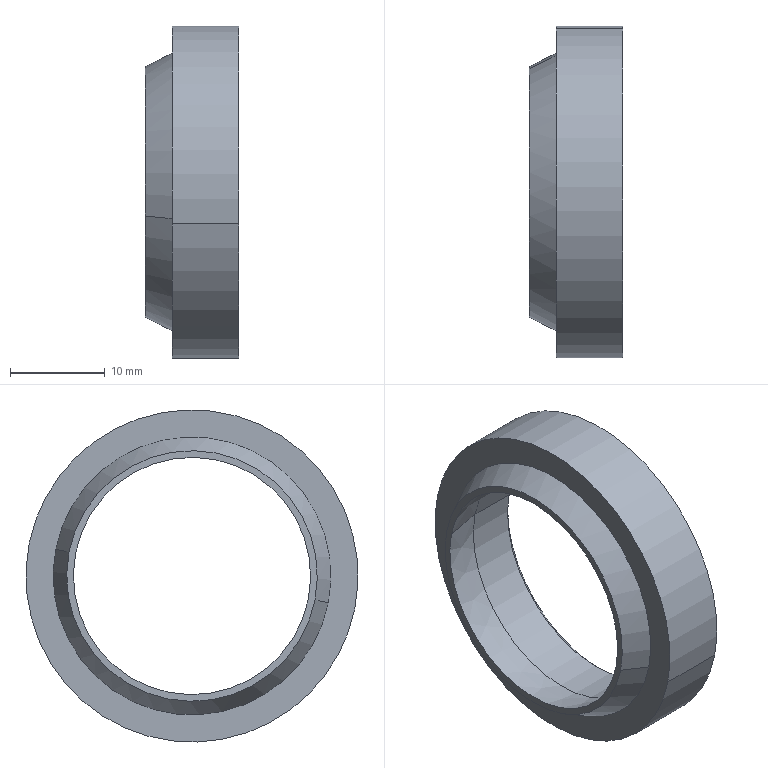Component | SolidWorks | GB_T10708.3-1989TypeBRubberDustSealFB20_35_7-1 | 1 solid | 13 faces | box 9.8 x 35 x 35 mm | volume 3185 mm3 | cone 6 | cylinder 4 | plane 3 | commonest cylinder face diameters 26.4 x2 35 x2
build123d program:
from build123d import *

# Parameters (mm, degrees)
CHAMFER1_SIZE = 0.5


with BuildPart() as part:
    # Sketch1 → Base-Revolve (revolve)
    with BuildSketch(Plane.XY, mode=Mode.PRIVATE) as base_revolve_sk:
        Polygon((12.5, 9.8), (13.2, 9.8), (14.633, 7), (17.5, 7), (17.5, 0), (13.2, 0), (13.2, 5.6), align=None)
    revolve(base_revolve_sk.sketch.rotate(Axis((0, 0, 0), (0, 1, 0)), 90), axis=Axis((0, 0, 0), (0, 1, 0)))

    # Chamfer1
    chamfer1_edges = [part.edges().sort_by_distance(p)[0] for p in [
        (0, 0, 13.2),
    ]]
    chamfer(chamfer1_edges, length=CHAMFER1_SIZE)


solid = part.part

# Placed as in the assembly
solid = solid.moved(Location((-465.364, 0, 0), (0, 0, 90)))
STEP:
#1=COLOUR_RGB('',0.7922,0.8196,0.9333);
#2=FILL_AREA_STYLE_COLOUR('',#1);
#3=FILL_AREA_STYLE('',(#2));
#4=SURFACE_STYLE_FILL_AREA(#3);
#5=SURFACE_SIDE_STYLE('',(#4));
#6=SURFACE_STYLE_USAGE(.BOTH.,#5);
#7=PRESENTATION_STYLE_ASSIGNMENT((#6));
#8=CARTESIAN_POINT('',(-18.341,-0.51,-0.09992));
#9=VERTEX_POINT('',#8);
#10=CARTESIAN_POINT('',(-18.341,0.51,0.09992));
#11=VERTEX_POINT('',#10);
#12=CARTESIAN_POINT('',(-18.341,0.,-0.));
#13=DIRECTION('',(1.,-0.,0.));
#14=DIRECTION('',(0.,0.9813,0.1923));
#15=AXIS2_PLACEMENT_3D('',#12,#13,#14);
#16=CIRCLE('',#15,0.5197);
#17=EDGE_CURVE('',#9,#11,#16,.T.);
#18=ORIENTED_EDGE('',*,*,#17,.F.);
#19=CARTESIAN_POINT('',(-18.321,-0.5293,-0.1037));
#20=VERTEX_POINT('',#19);
#21=CARTESIAN_POINT('',(-18.341,-0.51,-0.09992));
#22=DIRECTION('',(0.7071,-0.6939,-0.136));
#23=VECTOR('',#22,39.37);
#24=LINE('',#21,#23);
#25=EDGE_CURVE('',#9,#20,#24,.T.);
#26=ORIENTED_EDGE('',*,*,#25,.T.);
#27=CARTESIAN_POINT('',(-18.321,0.5293,0.1037));
#28=VERTEX_POINT('',#27);
#29=CARTESIAN_POINT('',(-18.321,0.,-0.));
#30=DIRECTION('',(-1.,0.,-0.));
#31=DIRECTION('',(0.,0.9813,0.1923));
#32=AXIS2_PLACEMENT_3D('',#29,#30,#31);
#33=CIRCLE('',#32,0.5394);
#34=EDGE_CURVE('',#28,#20,#33,.T.);
#35=ORIENTED_EDGE('',*,*,#34,.F.);
#36=CARTESIAN_POINT('',(-18.341,0.51,0.09992));
#37=DIRECTION('',(0.7071,0.6939,0.136));
#38=VECTOR('',#37,39.37);
#39=LINE('',#36,#38);
#40=EDGE_CURVE('',#11,#28,#39,.T.);
#41=ORIENTED_EDGE('',*,*,#40,.F.);
#42=EDGE_LOOP('',(#18,#26,#35,#41));
#43=FACE_OUTER_BOUND('',#42,.T.);
#44=CARTESIAN_POINT('',(-18.341,0.,-0.));
#45=DIRECTION('',(1.,-0.,0.));
#46=DIRECTION('',(0.,0.9813,0.1923));
#47=AXIS2_PLACEMENT_3D('',#44,#45,#46);
#48=CONICAL_SURFACE('',#47,0.5197,0.7854);
#49=ADVANCED_FACE('',(#43),#48,.F.);
#50=CARTESIAN_POINT('',(-18.542,-0.51,-0.09992));
#51=VERTEX_POINT('',#50);
#52=CARTESIAN_POINT('',(-18.542,0.51,0.09992));
#53=VERTEX_POINT('',#52);
#54=CARTESIAN_POINT('',(-18.542,0.,-0.));
#55=DIRECTION('',(1.,-0.,0.));
#56=DIRECTION('',(0.,0.9813,0.1923));
#57=AXIS2_PLACEMENT_3D('',#54,#55,#56);
#58=CIRCLE('',#57,0.5197);
#59=EDGE_CURVE('',#51,#53,#58,.T.);
#60=ORIENTED_EDGE('',*,*,#59,.F.);
#61=CARTESIAN_POINT('',(-18.321,-0.51,-0.09992));
#62=DIRECTION('',(1.,-0.,0.));
#63=VECTOR('',#62,39.37);
#64=LINE('',#61,#63);
#65=EDGE_CURVE('',#51,#9,#64,.T.);
#66=ORIENTED_EDGE('',*,*,#65,.T.);
#67=ORIENTED_EDGE('',*,*,#17,.T.);
#68=CARTESIAN_POINT('',(-18.321,0.51,0.09992));
#69=DIRECTION('',(1.,-0.,0.));
#70=VECTOR('',#69,39.37);
#71=LINE('',#68,#70);
#72=EDGE_CURVE('',#53,#11,#71,.T.);
#73=ORIENTED_EDGE('',*,*,#72,.F.);
#74=EDGE_LOOP('',(#60,#66,#67,#73));
#75=FACE_OUTER_BOUND('',#74,.T.);
#76=CARTESIAN_POINT('',(-18.321,0.,-0.));
#77=DIRECTION('',(1.,-0.,0.));
#78=DIRECTION('',(0.,0.9813,0.1923));
#79=AXIS2_PLACEMENT_3D('',#76,#77,#78);
#80=CYLINDRICAL_SURFACE('',#79,0.5197);
#81=ADVANCED_FACE('',(#75),#80,.F.);
#82=CARTESIAN_POINT('',(-18.597,0.6761,0.1325));
#83=VERTEX_POINT('',#82);
#84=CARTESIAN_POINT('',(-18.597,-0.6761,-0.1325));
#85=VERTEX_POINT('',#84);
#86=CARTESIAN_POINT('',(-18.597,0.,-0.));
#87=DIRECTION('',(1.,-0.,0.));
#88=DIRECTION('',(0.,0.9813,0.1923));
#89=AXIS2_PLACEMENT_3D('',#86,#87,#88);
#90=CIRCLE('',#89,0.689);
#91=EDGE_CURVE('',#83,#85,#90,.T.);
#92=ORIENTED_EDGE('',*,*,#91,.T.);
#93=CARTESIAN_POINT('',(-18.321,-0.6761,-0.1325));
#94=VERTEX_POINT('',#93);
#95=CARTESIAN_POINT('',(-18.321,-0.6761,-0.1325));
#96=DIRECTION('',(1.,-0.,0.));
#97=VECTOR('',#96,39.37);
#98=LINE('',#95,#97);
#99=EDGE_CURVE('',#85,#94,#98,.T.);
#100=ORIENTED_EDGE('',*,*,#99,.T.);
#101=CARTESIAN_POINT('',(-18.321,0.6761,0.1325));
#102=VERTEX_POINT('',#101);
#103=CARTESIAN_POINT('',(-18.321,0.,-0.));
#104=DIRECTION('',(1.,-0.,0.));
#105=DIRECTION('',(0.,0.9813,0.1923));
#106=AXIS2_PLACEMENT_3D('',#103,#104,#105);
#107=CIRCLE('',#106,0.689);
#108=EDGE_CURVE('',#102,#94,#107,.T.);
#109=ORIENTED_EDGE('',*,*,#108,.F.);
#110=CARTESIAN_POINT('',(-18.321,0.6761,0.1325));
#111=DIRECTION('',(1.,-0.,0.));
#112=VECTOR('',#111,39.37);
#113=LINE('',#110,#112);
#114=EDGE_CURVE('',#83,#102,#113,.T.);
#115=ORIENTED_EDGE('',*,*,#114,.F.);
#116=EDGE_LOOP('',(#92,#100,#109,#115));
#117=FACE_OUTER_BOUND('',#116,.T.);
#118=CARTESIAN_POINT('',(-18.321,0.,-0.));
#119=DIRECTION('',(1.,-0.,0.));
#120=DIRECTION('',(0.,0.9813,0.1923));
#121=AXIS2_PLACEMENT_3D('',#118,#119,#120);
#122=CYLINDRICAL_SURFACE('',#121,0.689);
#123=ADVANCED_FACE('',(#117),#122,.T.);
#124=CARTESIAN_POINT('',(-18.707,0.51,0.09992));
#125=VERTEX_POINT('',#124);
#126=CARTESIAN_POINT('',(-18.707,-0.51,-0.09992));
#127=VERTEX_POINT('',#126);
#128=CARTESIAN_POINT('',(-18.707,0.,-0.));
#129=DIRECTION('',(1.,-0.,0.));
#130=DIRECTION('',(0.,0.9813,0.1923));
#131=AXIS2_PLACEMENT_3D('',#128,#129,#130);
#132=CIRCLE('',#131,0.5197);
#133=EDGE_CURVE('',#125,#127,#132,.T.);
#134=ORIENTED_EDGE('',*,*,#133,.T.);
#135=CARTESIAN_POINT('',(-18.597,-0.5654,-0.1108));
#136=VERTEX_POINT('',#135);
#137=CARTESIAN_POINT('',(-18.597,-0.5654,-0.1108));
#138=DIRECTION('',(0.8901,-0.4472,-0.08761));
#139=VECTOR('',#138,39.37);
#140=LINE('',#137,#139);
#141=EDGE_CURVE('',#127,#136,#140,.T.);
#142=ORIENTED_EDGE('',*,*,#141,.T.);
#143=CARTESIAN_POINT('',(-18.597,0.5654,0.1108));
#144=VERTEX_POINT('',#143);
#145=CARTESIAN_POINT('',(-18.597,0.,-0.));
#146=DIRECTION('',(1.,-0.,0.));
#147=DIRECTION('',(0.,0.9813,0.1923));
#148=AXIS2_PLACEMENT_3D('',#145,#146,#147);
#149=CIRCLE('',#148,0.5761);
#150=EDGE_CURVE('',#144,#136,#149,.T.);
#151=ORIENTED_EDGE('',*,*,#150,.F.);
#152=CARTESIAN_POINT('',(-18.597,0.5654,0.1108));
#153=DIRECTION('',(0.8901,0.4472,0.08761));
#154=VECTOR('',#153,39.37);
#155=LINE('',#152,#154);
#156=EDGE_CURVE('',#125,#144,#155,.T.);
#157=ORIENTED_EDGE('',*,*,#156,.F.);
#158=EDGE_LOOP('',(#134,#142,#151,#157));
#159=FACE_OUTER_BOUND('',#158,.T.);
#160=CARTESIAN_POINT('',(-18.597,0.,-0.));
#161=DIRECTION('',(1.,-0.,0.));
#162=DIRECTION('',(0.,0.9813,0.1923));
#163=AXIS2_PLACEMENT_3D('',#160,#161,#162);
#164=CONICAL_SURFACE('',#163,0.5761,0.4731);
#165=ADVANCED_FACE('',(#159),#164,.T.);
#166=CARTESIAN_POINT('',(-18.707,-0.4829,-0.09462));
#167=VERTEX_POINT('',#166);
#168=CARTESIAN_POINT('',(-18.707,0.4829,0.09462));
#169=VERTEX_POINT('',#168);
#170=CARTESIAN_POINT('',(-18.707,0.,-0.));
#171=DIRECTION('',(1.,-0.,0.));
#172=DIRECTION('',(0.,0.9813,0.1923));
#173=AXIS2_PLACEMENT_3D('',#170,#171,#172);
#174=CIRCLE('',#173,0.4921);
#175=EDGE_CURVE('',#167,#169,#174,.T.);
#176=ORIENTED_EDGE('',*,*,#175,.F.);
#177=CARTESIAN_POINT('',(-18.707,-0.4829,-0.09462));
#178=DIRECTION('',(0.9864,-0.1613,-0.03161));
#179=VECTOR('',#178,39.37);
#180=LINE('',#177,#179);
#181=EDGE_CURVE('',#167,#51,#180,.T.);
#182=ORIENTED_EDGE('',*,*,#181,.T.);
#183=ORIENTED_EDGE('',*,*,#59,.T.);
#184=CARTESIAN_POINT('',(-18.707,0.4829,0.09462));
#185=DIRECTION('',(0.9864,0.1613,0.03161));
#186=VECTOR('',#185,39.37);
#187=LINE('',#184,#186);
#188=EDGE_CURVE('',#169,#53,#187,.T.);
#189=ORIENTED_EDGE('',*,*,#188,.F.);
#190=EDGE_LOOP('',(#176,#182,#183,#189));
#191=FACE_OUTER_BOUND('',#190,.T.);
#192=CARTESIAN_POINT('',(-18.707,0.,-0.));
#193=DIRECTION('',(1.,-0.,0.));
#194=DIRECTION('',(0.,0.9813,0.1923));
#195=AXIS2_PLACEMENT_3D('',#192,#193,#194);
#196=CONICAL_SURFACE('',#195,0.4921,0.1651);
#197=ADVANCED_FACE('',(#191),#196,.F.);
#198=ORIENTED_EDGE('',*,*,#181,.F.);
#199=CARTESIAN_POINT('',(-18.707,0.,-0.));
#200=DIRECTION('',(1.,-0.,0.));
#201=DIRECTION('',(0.,0.9813,0.1923));
#202=AXIS2_PLACEMENT_3D('',#199,#200,#201);
#203=CIRCLE('',#202,0.4921);
#204=EDGE_CURVE('',#169,#167,#203,.T.);
#205=ORIENTED_EDGE('',*,*,#204,.F.);
#206=ORIENTED_EDGE('',*,*,#188,.T.);
#207=CARTESIAN_POINT('',(-18.542,0.,-0.));
#208=DIRECTION('',(1.,-0.,0.));
#209=DIRECTION('',(0.,0.9813,0.1923));
#210=AXIS2_PLACEMENT_3D('',#207,#208,#209);
#211=CIRCLE('',#210,0.5197);
#212=EDGE_CURVE('',#53,#51,#211,.T.);
#213=ORIENTED_EDGE('',*,*,#212,.T.);
#214=EDGE_LOOP('',(#198,#205,#206,#213));
#215=FACE_OUTER_BOUND('',#214,.T.);
#216=CARTESIAN_POINT('',(-18.707,0.,-0.));
#217=DIRECTION('',(1.,-0.,0.));
#218=DIRECTION('',(0.,0.9813,0.1923));
#219=AXIS2_PLACEMENT_3D('',#216,#217,#218);
#220=CONICAL_SURFACE('',#219,0.4921,0.1651);
#221=ADVANCED_FACE('',(#215),#220,.F.);
#222=ORIENTED_EDGE('',*,*,#204,.T.);
#223=ORIENTED_EDGE('',*,*,#175,.T.);
#224=EDGE_LOOP('',(#222,#223));
#225=FACE_BOUND('',#224,.T.);
#226=ORIENTED_EDGE('',*,*,#133,.F.);
#227=CARTESIAN_POINT('',(-18.707,0.,-0.));
#228=DIRECTION('',(1.,-0.,0.));
#229=DIRECTION('',(0.,0.9813,0.1923));
#230=AXIS2_PLACEMENT_3D('',#227,#228,#229);
#231=CIRCLE('',#230,0.5197);
#232=EDGE_CURVE('',#127,#125,#231,.T.);
#233=ORIENTED_EDGE('',*,*,#232,.F.);
#234=EDGE_LOOP('',(#226,#233));
#235=FACE_OUTER_BOUND('',#234,.T.);
#236=CARTESIAN_POINT('',(-18.707,-0.09462,0.4829));
#237=DIRECTION('',(-1.,0.,-0.));
#238=DIRECTION('',(-0.,-0.9813,-0.1923));
#239=AXIS2_PLACEMENT_3D('',#236,#237,#238);
#240=PLANE('',#239);
#241=ADVANCED_FACE('',(#225,#235),#240,.T.);
#242=ORIENTED_EDGE('',*,*,#141,.F.);
#243=ORIENTED_EDGE('',*,*,#232,.T.);
#244=ORIENTED_EDGE('',*,*,#156,.T.);
#245=CARTESIAN_POINT('',(-18.597,0.,-0.));
#246=DIRECTION('',(1.,-0.,0.));
#247=DIRECTION('',(0.,0.9813,0.1923));
#248=AXIS2_PLACEMENT_3D('',#245,#246,#247);
#249=CIRCLE('',#248,0.5761);
#250=EDGE_CURVE('',#136,#144,#249,.T.);
#251=ORIENTED_EDGE('',*,*,#250,.F.);
#252=EDGE_LOOP('',(#242,#243,#244,#251));
#253=FACE_OUTER_BOUND('',#252,.T.);
#254=CARTESIAN_POINT('',(-18.597,0.,-0.));
#255=DIRECTION('',(1.,-0.,0.));
#256=DIRECTION('',(0.,0.9813,0.1923));
#257=AXIS2_PLACEMENT_3D('',#254,#255,#256);
#258=CONICAL_SURFACE('',#257,0.5761,0.4731);
#259=ADVANCED_FACE('',(#253),#258,.T.);
#260=ORIENTED_EDGE('',*,*,#150,.T.);
#261=ORIENTED_EDGE('',*,*,#250,.T.);
#262=EDGE_LOOP('',(#260,#261));
#263=FACE_BOUND('',#262,.T.);
#264=ORIENTED_EDGE('',*,*,#91,.F.);
#265=CARTESIAN_POINT('',(-18.597,0.,-0.));
#266=DIRECTION('',(1.,-0.,0.));
#267=DIRECTION('',(0.,0.9813,0.1923));
#268=AXIS2_PLACEMENT_3D('',#265,#266,#267);
#269=CIRCLE('',#268,0.689);
#270=EDGE_CURVE('',#85,#83,#269,.T.);
#271=ORIENTED_EDGE('',*,*,#270,.F.);
#272=EDGE_LOOP('',(#264,#271));
#273=FACE_OUTER_BOUND('',#272,.T.);
#274=CARTESIAN_POINT('',(-18.597,-0.1108,0.5654));
#275=DIRECTION('',(-1.,0.,-0.));
#276=DIRECTION('',(-0.,-0.9813,-0.1923));
#277=AXIS2_PLACEMENT_3D('',#274,#275,#276);
#278=PLANE('',#277);
#279=ADVANCED_FACE('',(#263,#273),#278,.T.);
#280=ORIENTED_EDGE('',*,*,#99,.F.);
#281=ORIENTED_EDGE('',*,*,#270,.T.);
#282=ORIENTED_EDGE('',*,*,#114,.T.);
#283=CARTESIAN_POINT('',(-18.321,0.,-0.));
#284=DIRECTION('',(1.,-0.,0.));
#285=DIRECTION('',(0.,0.9813,0.1923));
#286=AXIS2_PLACEMENT_3D('',#283,#284,#285);
#287=CIRCLE('',#286,0.689);
#288=EDGE_CURVE('',#94,#102,#287,.T.);
#289=ORIENTED_EDGE('',*,*,#288,.F.);
#290=EDGE_LOOP('',(#280,#281,#282,#289));
#291=FACE_OUTER_BOUND('',#290,.T.);
#292=CARTESIAN_POINT('',(-18.321,0.,-0.));
#293=DIRECTION('',(1.,-0.,0.));
#294=DIRECTION('',(0.,0.9813,0.1923));
#295=AXIS2_PLACEMENT_3D('',#292,#293,#294);
#296=CYLINDRICAL_SURFACE('',#295,0.689);
#297=ADVANCED_FACE('',(#291),#296,.T.);
#298=ORIENTED_EDGE('',*,*,#34,.T.);
#299=CARTESIAN_POINT('',(-18.321,0.,-0.));
#300=DIRECTION('',(-1.,0.,-0.));
#301=DIRECTION('',(0.,0.9813,0.1923));
#302=AXIS2_PLACEMENT_3D('',#299,#300,#301);
#303=CIRCLE('',#302,0.5394);
#304=EDGE_CURVE('',#20,#28,#303,.T.);
#305=ORIENTED_EDGE('',*,*,#304,.T.);
#306=EDGE_LOOP('',(#298,#305));
#307=FACE_BOUND('',#306,.T.);
#308=ORIENTED_EDGE('',*,*,#108,.T.);
#309=ORIENTED_EDGE('',*,*,#288,.T.);
#310=EDGE_LOOP('',(#308,#309));
#311=FACE_OUTER_BOUND('',#310,.T.);
#312=CARTESIAN_POINT('',(-18.321,-0.1325,0.6761));
#313=DIRECTION('',(1.,-0.,0.));
#314=DIRECTION('',(0.,0.9813,0.1923));
#315=AXIS2_PLACEMENT_3D('',#312,#313,#314);
#316=PLANE('',#315);
#317=ADVANCED_FACE('',(#307,#311),#316,.T.);
#318=ORIENTED_EDGE('',*,*,#65,.F.);
#319=ORIENTED_EDGE('',*,*,#212,.F.);
#320=ORIENTED_EDGE('',*,*,#72,.T.);
#321=CARTESIAN_POINT('',(-18.341,0.,-0.));
#322=DIRECTION('',(1.,-0.,0.));
#323=DIRECTION('',(0.,0.9813,0.1923));
#324=AXIS2_PLACEMENT_3D('',#321,#322,#323);
#325=CIRCLE('',#324,0.5197);
#326=EDGE_CURVE('',#11,#9,#325,.T.);
#327=ORIENTED_EDGE('',*,*,#326,.T.);
#328=EDGE_LOOP('',(#318,#319,#320,#327));
#329=FACE_OUTER_BOUND('',#328,.T.);
#330=CARTESIAN_POINT('',(-18.321,0.,-0.));
#331=DIRECTION('',(1.,-0.,0.));
#332=DIRECTION('',(0.,0.9813,0.1923));
#333=AXIS2_PLACEMENT_3D('',#330,#331,#332);
#334=CYLINDRICAL_SURFACE('',#333,0.5197);
#335=ADVANCED_FACE('',(#329),#334,.F.);
#336=ORIENTED_EDGE('',*,*,#25,.F.);
#337=ORIENTED_EDGE('',*,*,#326,.F.);
#338=ORIENTED_EDGE('',*,*,#40,.T.);
#339=ORIENTED_EDGE('',*,*,#304,.F.);
#340=EDGE_LOOP('',(#336,#337,#338,#339));
#341=FACE_OUTER_BOUND('',#340,.T.);
#342=CARTESIAN_POINT('',(-18.341,0.,-0.));
#343=DIRECTION('',(1.,-0.,0.));
#344=DIRECTION('',(0.,0.9813,0.1923));
#345=AXIS2_PLACEMENT_3D('',#342,#343,#344);
#346=CONICAL_SURFACE('',#345,0.5197,0.7854);
#347=ADVANCED_FACE('',(#341),#346,.F.);
#348=CLOSED_SHELL('',(#49,#81,#123,#165,#197,#221,#241,#259,#279,#297,#317,#335,#347));
#349=MANIFOLD_SOLID_BREP('',#348);
#350=STYLED_ITEM('',(#7),#349);
#351=(LENGTH_UNIT()NAMED_UNIT(*)SI_UNIT($,.METRE.));
#352=LENGTH_MEASURE_WITH_UNIT(LENGTH_MEASURE(0.0254),#351);
#353=DIMENSIONAL_EXPONENTS(1.,0.,0.,0.,0.,0.,0.);
#354=(CONVERSION_BASED_UNIT('',#352)LENGTH_UNIT()NAMED_UNIT(#353));
#355=UNCERTAINTY_MEASURE_WITH_UNIT(LENGTH_MEASURE(0.00001),#354,'','');
#356=(NAMED_UNIT(*)PLANE_ANGLE_UNIT()SI_UNIT($,.RADIAN.));
#357=(NAMED_UNIT(*)SI_UNIT($,.STERADIAN.)SOLID_ANGLE_UNIT());
#358=(GEOMETRIC_REPRESENTATION_CONTEXT(3)GLOBAL_UNCERTAINTY_ASSIGNED_CONTEXT((#355))GLOBAL_UNIT_ASSIGNED_CONTEXT((#354,#356,#357))REPRESENTATION_CONTEXT('',''));
#359=MECHANICAL_DESIGN_GEOMETRIC_PRESENTATION_REPRESENTATION('',(#350),#358);
#360=PRESENTATION_LAYER_ASSIGNMENT('','',(#350));
#361=CARTESIAN_POINT('',(0.,0.,0.));
#362=DIRECTION('',(0.,0.,1.));
#363=DIRECTION('',(1.,0.,0.));
#364=AXIS2_PLACEMENT_3D('',#361,#362,#363);
#365=(LENGTH_UNIT()NAMED_UNIT(*)SI_UNIT($,.METRE.));
#366=LENGTH_MEASURE_WITH_UNIT(LENGTH_MEASURE(0.0254),#365);
#367=DIMENSIONAL_EXPONENTS(1.,0.,0.,0.,0.,0.,0.);
#368=(CONVERSION_BASED_UNIT('',#366)LENGTH_UNIT()NAMED_UNIT(#367));
#369=UNCERTAINTY_MEASURE_WITH_UNIT(LENGTH_MEASURE(0.00001),#368,'','');
#370=(NAMED_UNIT(*)PLANE_ANGLE_UNIT()SI_UNIT($,.RADIAN.));
#371=(NAMED_UNIT(*)SI_UNIT($,.STERADIAN.)SOLID_ANGLE_UNIT());
#372=(GEOMETRIC_REPRESENTATION_CONTEXT(3)GLOBAL_UNCERTAINTY_ASSIGNED_CONTEXT((#369))GLOBAL_UNIT_ASSIGNED_CONTEXT((#368,#370,#371))REPRESENTATION_CONTEXT('',''));
#373=ADVANCED_BREP_SHAPE_REPRESENTATION('',(#349,#364),#372);